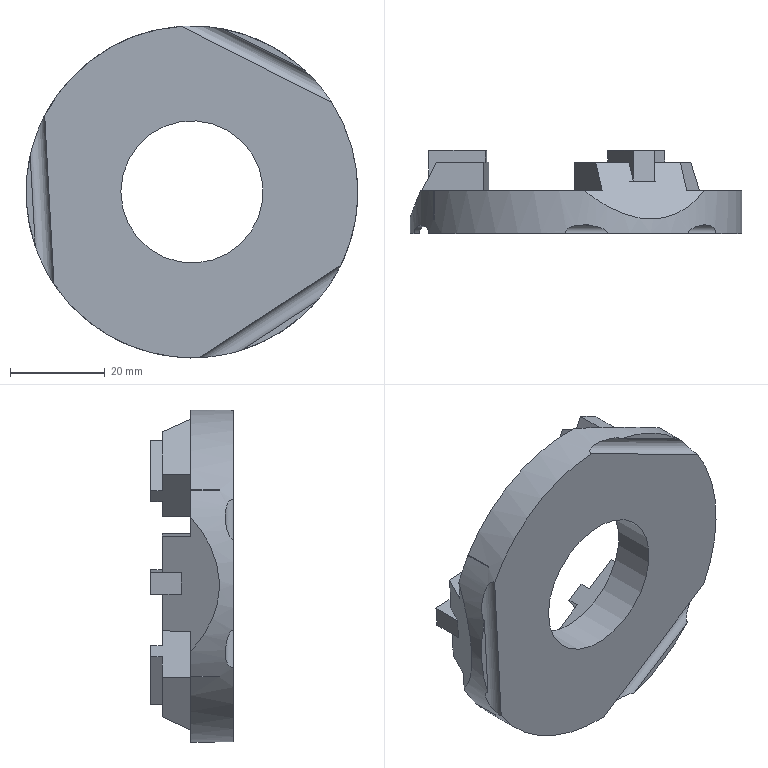Component | NX | DRIVE_FLANGE | 1 solid | 60 faces | volume 32117 mm3 | plane 55 | cylinder 5 | commonest cylinder face diameters 3.518 x3 70 x1 30 x1